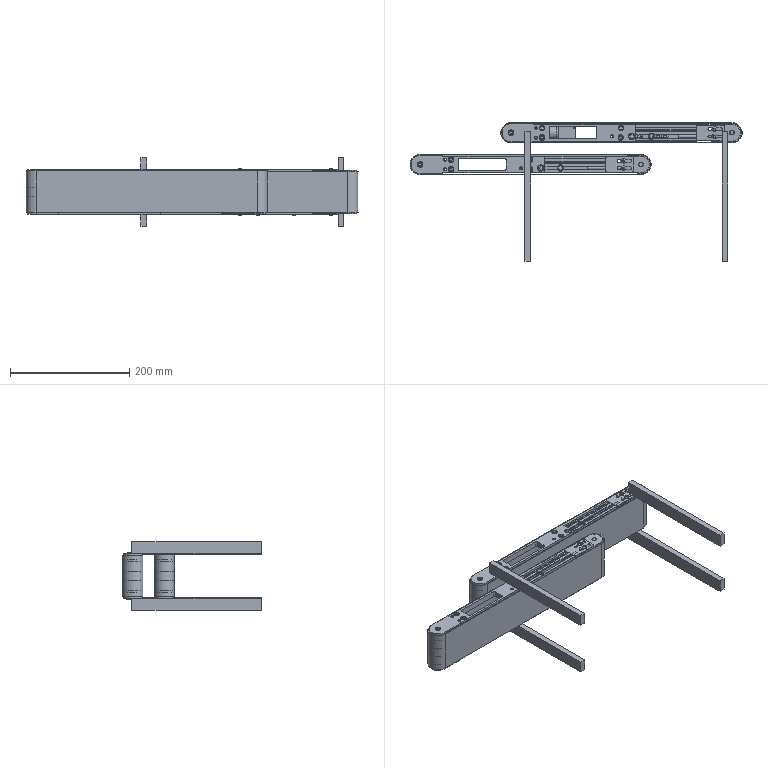Assembly | NX | mm | 13 component files | 13 solids | 2099 faces | box 555.99 x 231.9 x 115 mm | volume 1132585 mm3 | plane 1441 | cylinder 404 | cone 232 | spline 16 | torus 6 | commonest cylinder face diameters 11.5 x40 4 x38 6 x30 9.5 x20 8.5 x20 4.4 x18 0.6 x16 10 x16
Bill of materials:
unnamed part 1 | 1 |  | Long, narrow multi-body frame with rounded ends. It has a faceted barrel-shaped roller at one end and a pair of smaller stacked rollers at the other, with pockets, a rectangular through-slot, rail-like grooves, and many small holes along the top.
unnamed part 2 | 6 |  | Hexagonal nut-shaped body with a central through-bore and a chamfered entry on one face. The edges on the opposite face are curved, consistent with a chamfer.
unnamed part 3 | 1 |  | The same kind of elongated frame-and-roller body as part-16f5..., plus four long, straight, rectangular-section bars. The bars stick out perpendicular to the frame, two near each end, forming a U-shaped or table-like layout.
unnamed part 4 | 1 |  | Thin, flat rectangular plate with rounded corners. Near each end, a hex-headed fastener-like body passes through it, with a rounded, faceted dome below the plate.
unnamed part 5 | 1 |  | Straight prismatic bar with a stadium (obround) cross-section: two flat parallel sides joined by semicircular ends, extruded to a constant length.
unnamed part 6 | 1 |  | Straight prismatic bar with a stadium (obround) cross-section: two flat parallel sides joined by semicircular ends, extruded to a constant length.
unnamed part 7 | 1 |  | Revolved body made of two cylindrical bosses whose axes meet at roughly a right angle, joined through conical or flared collars. One boss has a through-bore, a small circumferential groove and a stepped flange; the other has a smaller through-bore.
unnamed part 8 | 1 |  | Compact body made of a cylindrical section, with a stepped smaller cylindrical spigot and a protruding round shaft at one end, joined through a thin flange ring to a box-shaped rectangular block at the other end. The block has two small rounded bosses at opposite corners of its end face.
Mates:
1. fix | CVSMB_b_g 1 component
2. fix | CVSMB_3_5_DC24_SCM_64_DA_m 1 component
3. fix | CVS__Nut-M6 1 component
4. fix | CVS__Nut-M6 2 component
5. fix | CVS__Nut-M6 3 component
6. fix | CVS__Nut-M6 4 component
7. fix | CVS__Nut-M6 5 component
8. fix | CVS__Nut-M6 6 component
9. fix | CVSMB_p 1 component
10. fix | CVSMB_70_370_H_b 1 component
11. fix | CVSMB_70_370_3_5_DC24_SCM_H_DA_l 1 component